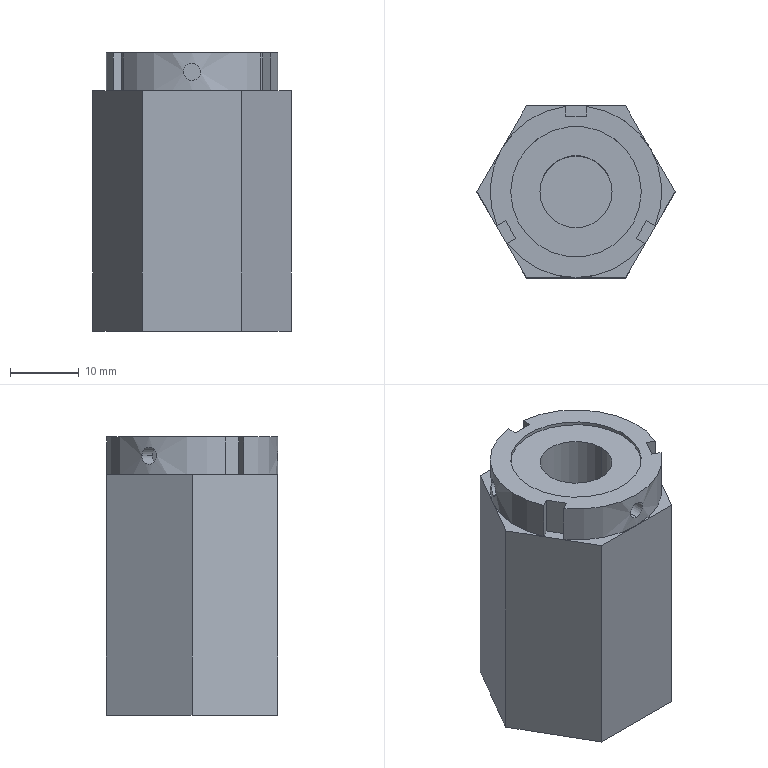CAM job | Mastercam | mm | 14 operations | part box 210 x 297 x 40.5
1. Facing | 20 - 63 平铣刀
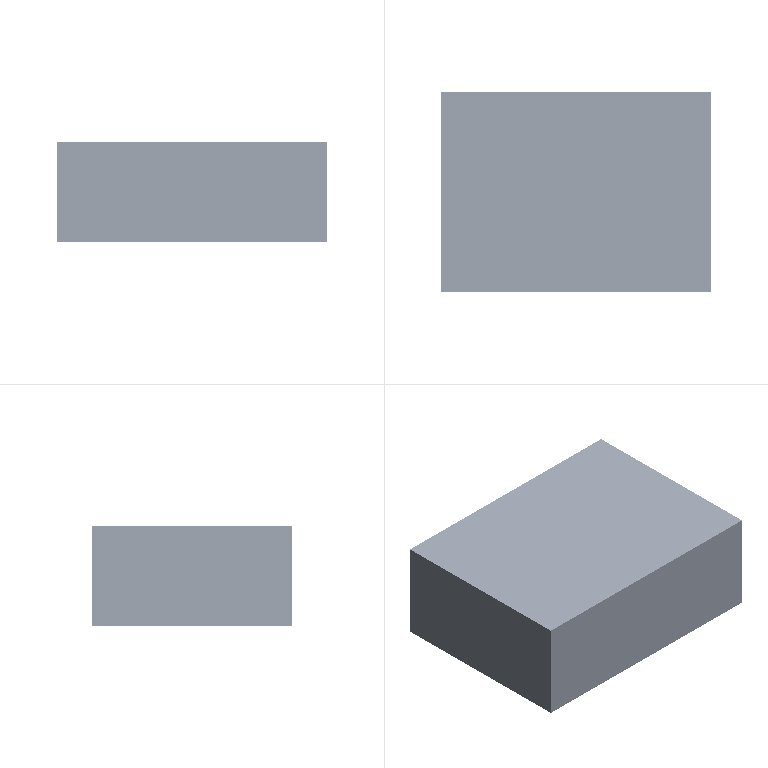2. Contour (Ramp) | 12 - 12 平铣刀
3. Contour (Ramp) | 12 - 12 平铣刀
4. Contour (2D) | 12 - 12 平铣刀
5. Contour (2D) | 12 - 12 平铣刀
6. Contour (Ramp) | 6 - 6 平铣刀
7. Contour (2D chamfer) | 7 - 4 倒角刀
8. Facing | 20 - 63 平铣刀
9. Contour (2D chamfer) | 7 - 4 倒角刀
10. Contour (2D) | 2 - 2 平铣刀
11. Contour (2D) | 2 - 2 平铣刀
12. Contour (2D chamfer) | 7 - 4 倒角刀
13. Drill/Counterbore | 7 - 4 倒角刀
14. Peck Drill | 1 - 2.5 钻头